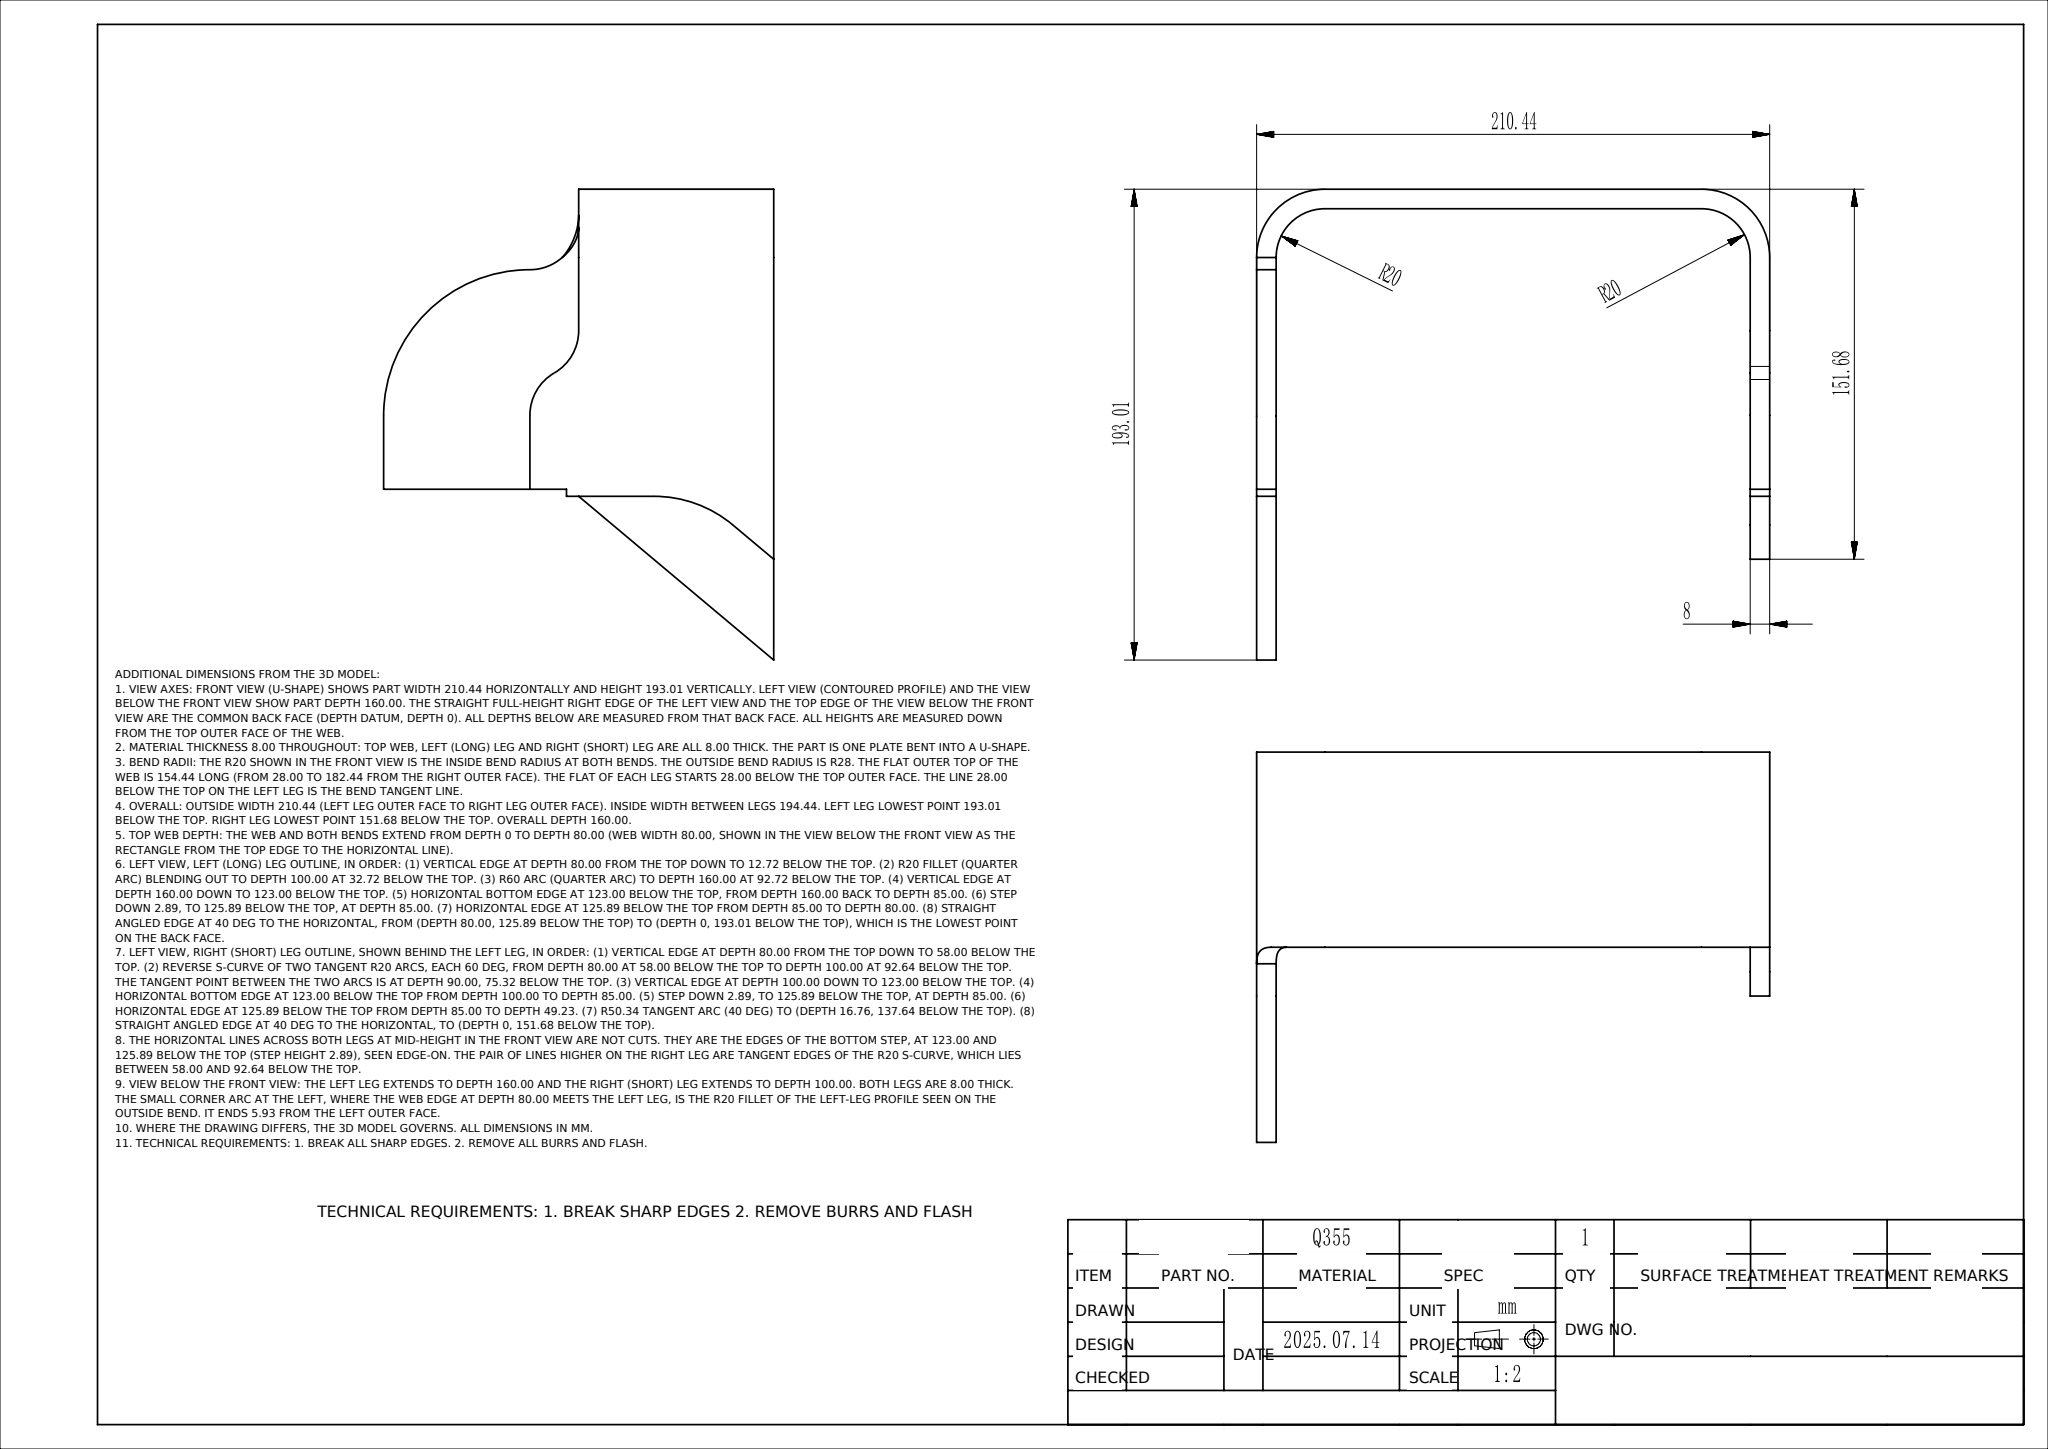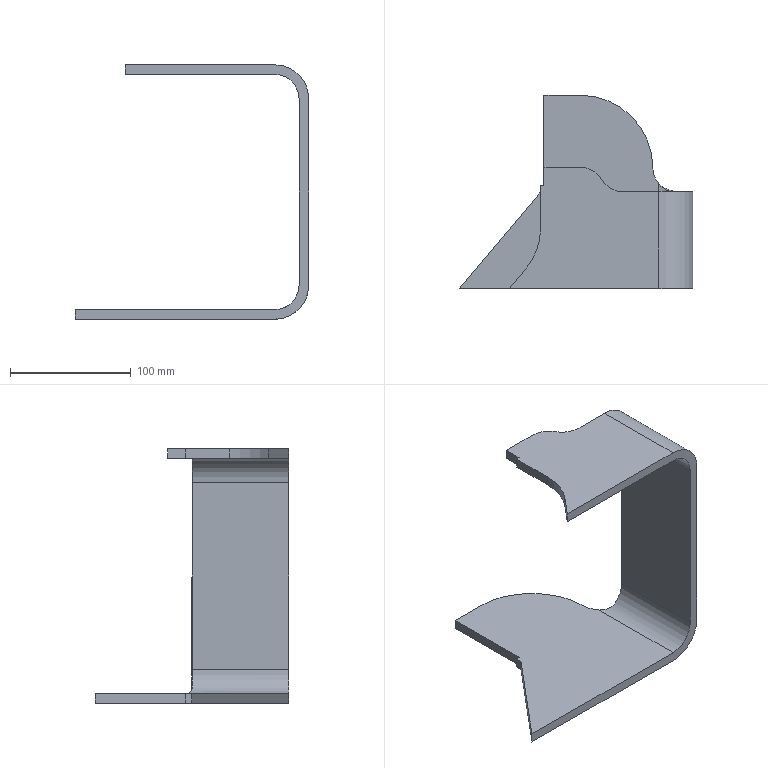Part | NX | mm | 1 solid | 28 faces | box 193.01 x 160 x 210.44 mm | volume 357331 mm3 | plane 18 | cylinder 9 | spline 1 | commonest cylinder face diameters 40 x5 56 x2 120 x1 100.67 x1
STEP:
#1=CARTESIAN_POINT('',(0.,0.,0.));
#2=DIRECTION('',(0.,0.,1.));
#3=DIRECTION('',(1.,0.,0.));
#4=AXIS2_PLACEMENT_3D('',#1,#2,#3);
#5=(LENGTH_UNIT()NAMED_UNIT(*)SI_UNIT(.MILLI.,.METRE.));
#6=UNCERTAINTY_MEASURE_WITH_UNIT(LENGTH_MEASURE(0.0508),#5,'','');
#7=(NAMED_UNIT(*)PLANE_ANGLE_UNIT()SI_UNIT($,.RADIAN.));
#8=PLANE_ANGLE_MEASURE_WITH_UNIT(PLANE_ANGLE_MEASURE(0.01745),#7);
#9=DIMENSIONAL_EXPONENTS(0.,0.,0.,0.,0.,0.,0.);
#10=(CONVERSION_BASED_UNIT('',#8)NAMED_UNIT(#9)PLANE_ANGLE_UNIT());
#11=(NAMED_UNIT(*)SI_UNIT($,.STERADIAN.)SOLID_ANGLE_UNIT());
#12=(GEOMETRIC_REPRESENTATION_CONTEXT(3)GLOBAL_UNCERTAINTY_ASSIGNED_CONTEXT((#6))GLOBAL_UNIT_ASSIGNED_CONTEXT((#5,#10,#11))REPRESENTATION_CONTEXT('',''));
#13=SHAPE_REPRESENTATION('',(#4),#12);
#14=CARTESIAN_POINT('',(123.,-85.,-28.));
#15=VERTEX_POINT('',#14);
#16=CARTESIAN_POINT('',(123.,-85.,-182.437));
#17=VERTEX_POINT('',#16);
#18=CARTESIAN_POINT('',(123.,-85.,131.244));
#19=DIRECTION('',(0.,0.,-1.));
#20=VECTOR('',#19,1.);
#21=LINE('',#18,#20);
#22=EDGE_CURVE('',#15,#17,#21,.T.);
#23=ORIENTED_EDGE('',*,*,#22,.F.);
#24=CARTESIAN_POINT('',(95.,-85.,0.));
#25=VERTEX_POINT('',#24);
#26=CARTESIAN_POINT('',(95.,-85.,-28.));
#27=DIRECTION('',(0.,1.,0.));
#28=DIRECTION('',(0.,0.,-1.));
#29=AXIS2_PLACEMENT_3D('',#26,#27,#28);
#30=CIRCLE('',#29,28.);
#31=EDGE_CURVE('',#25,#15,#30,.T.);
#32=ORIENTED_EDGE('',*,*,#31,.F.);
#33=CARTESIAN_POINT('',(-28.681,-85.,0.));
#34=VERTEX_POINT('',#33);
#35=CARTESIAN_POINT('',(-28.681,-85.,0.));
#36=DIRECTION('',(1.,0.,0.));
#37=VECTOR('',#36,1.);
#38=LINE('',#35,#37);
#39=EDGE_CURVE('',#34,#25,#38,.T.);
#40=ORIENTED_EDGE('',*,*,#39,.F.);
#41=CARTESIAN_POINT('',(-28.681,-85.,-8.));
#42=VERTEX_POINT('',#41);
#43=CARTESIAN_POINT('',(-28.681,-85.,-8.));
#44=DIRECTION('',(0.,0.,1.));
#45=VECTOR('',#44,1.);
#46=LINE('',#43,#45);
#47=EDGE_CURVE('',#42,#34,#46,.T.);
#48=ORIENTED_EDGE('',*,*,#47,.F.);
#49=CARTESIAN_POINT('',(95.,-85.,-8.));
#50=VERTEX_POINT('',#49);
#51=CARTESIAN_POINT('',(-28.681,-85.,-8.));
#52=DIRECTION('',(1.,0.,0.));
#53=VECTOR('',#52,1.);
#54=LINE('',#51,#53);
#55=EDGE_CURVE('',#42,#50,#54,.T.);
#56=ORIENTED_EDGE('',*,*,#55,.T.);
#57=CARTESIAN_POINT('',(115.,-85.,-28.));
#58=VERTEX_POINT('',#57);
#59=CARTESIAN_POINT('',(95.,-85.,-28.));
#60=DIRECTION('',(0.,1.,0.));
#61=DIRECTION('',(0.,0.,1.));
#62=AXIS2_PLACEMENT_3D('',#59,#60,#61);
#63=CIRCLE('',#62,20.);
#64=EDGE_CURVE('',#50,#58,#63,.T.);
#65=ORIENTED_EDGE('',*,*,#64,.T.);
#66=CARTESIAN_POINT('',(115.,-85.,-182.437));
#67=VERTEX_POINT('',#66);
#68=CARTESIAN_POINT('',(115.,-85.,131.244));
#69=DIRECTION('',(0.,0.,-1.));
#70=VECTOR('',#69,1.);
#71=LINE('',#68,#70);
#72=EDGE_CURVE('',#58,#67,#71,.T.);
#73=ORIENTED_EDGE('',*,*,#72,.T.);
#74=CARTESIAN_POINT('',(95.,-85.,-202.437));
#75=VERTEX_POINT('',#74);
#76=CARTESIAN_POINT('',(95.,-85.,-182.437));
#77=DIRECTION('',(0.,1.,0.));
#78=DIRECTION('',(1.,0.,0.));
#79=AXIS2_PLACEMENT_3D('',#76,#77,#78);
#80=CIRCLE('',#79,20.);
#81=EDGE_CURVE('',#67,#75,#80,.T.);
#82=ORIENTED_EDGE('',*,*,#81,.T.);
#83=CARTESIAN_POINT('',(-70.014,-85.,-202.437));
#84=VERTEX_POINT('',#83);
#85=CARTESIAN_POINT('',(444.244,-85.,-202.437));
#86=DIRECTION('',(-1.,0.,-0.));
#87=VECTOR('',#86,1.);
#88=LINE('',#85,#87);
#89=EDGE_CURVE('',#75,#84,#88,.T.);
#90=ORIENTED_EDGE('',*,*,#89,.T.);
#91=CARTESIAN_POINT('',(-70.014,-85.,-210.437));
#92=VERTEX_POINT('',#91);
#93=CARTESIAN_POINT('',(-70.014,-85.,-202.437));
#94=DIRECTION('',(0.,0.,-1.));
#95=VECTOR('',#94,1.);
#96=LINE('',#93,#95);
#97=EDGE_CURVE('',#84,#92,#96,.T.);
#98=ORIENTED_EDGE('',*,*,#97,.T.);
#99=CARTESIAN_POINT('',(95.,-85.,-210.437));
#100=VERTEX_POINT('',#99);
#101=CARTESIAN_POINT('',(444.244,-85.,-210.437));
#102=DIRECTION('',(-1.,0.,-0.));
#103=VECTOR('',#102,1.);
#104=LINE('',#101,#103);
#105=EDGE_CURVE('',#100,#92,#104,.T.);
#106=ORIENTED_EDGE('',*,*,#105,.F.);
#107=CARTESIAN_POINT('',(95.,-85.,-182.437));
#108=DIRECTION('',(0.,1.,0.));
#109=DIRECTION('',(-1.,0.,-0.));
#110=AXIS2_PLACEMENT_3D('',#107,#108,#109);
#111=CIRCLE('',#110,28.);
#112=EDGE_CURVE('',#17,#100,#111,.T.);
#113=ORIENTED_EDGE('',*,*,#112,.F.);
#114=EDGE_LOOP('',(#23,#32,#40,#48,#56,#65,#73,#82,#90,#98,#106,#113));
#115=FACE_OUTER_BOUND('',#114,.T.);
#116=CARTESIAN_POINT('',(444.244,-85.,-202.437));
#117=DIRECTION('',(-0.,-1.,-0.));
#118=DIRECTION('',(-1.,0.,-0.));
#119=AXIS2_PLACEMENT_3D('',#116,#117,#118);
#120=PLANE('',#119);
#121=ADVANCED_FACE('',(#115),#120,.T.);
#122=CARTESIAN_POINT('',(123.,-5.,-182.437));
#123=VERTEX_POINT('',#122);
#124=CARTESIAN_POINT('',(123.,-5.,-28.));
#125=VERTEX_POINT('',#124);
#126=CARTESIAN_POINT('',(123.,-5.,-222.997));
#127=DIRECTION('',(-0.,-0.,1.));
#128=VECTOR('',#127,1.);
#129=LINE('',#126,#128);
#130=EDGE_CURVE('',#123,#125,#129,.T.);
#131=ORIENTED_EDGE('',*,*,#130,.T.);
#132=CARTESIAN_POINT('',(123.,50.,-28.));
#133=DIRECTION('',(0.,-1.,-0.));
#134=VECTOR('',#133,1.);
#135=LINE('',#132,#134);
#136=EDGE_CURVE('',#125,#15,#135,.T.);
#137=ORIENTED_EDGE('',*,*,#136,.T.);
#138=ORIENTED_EDGE('',*,*,#22,.T.);
#139=CARTESIAN_POINT('',(123.,45.151,-182.437));
#140=DIRECTION('',(0.,1.,0.));
#141=VECTOR('',#140,1.);
#142=LINE('',#139,#141);
#143=EDGE_CURVE('',#17,#123,#142,.T.);
#144=ORIENTED_EDGE('',*,*,#143,.T.);
#145=EDGE_LOOP('',(#131,#137,#138,#144));
#146=FACE_OUTER_BOUND('',#145,.T.);
#147=CARTESIAN_POINT('',(123.,-35.915,155.787));
#148=DIRECTION('',(-1.,0.,-0.));
#149=DIRECTION('',(-0.,0.,1.));
#150=AXIS2_PLACEMENT_3D('',#147,#148,#149);
#151=PLANE('',#150);
#152=ADVANCED_FACE('',(#146),#151,.F.);
#153=CARTESIAN_POINT('',(90.003,15.,-210.437));
#154=VERTEX_POINT('',#153);
#155=CARTESIAN_POINT('',(95.,1.774,-210.437));
#156=VERTEX_POINT('',#155);
#157=CARTESIAN_POINT('',(110.003,15.,-210.437));
#158=DIRECTION('',(-0.,0.,1.));
#159=DIRECTION('',(1.,0.,0.));
#160=AXIS2_PLACEMENT_3D('',#157,#158,#159);
#161=CIRCLE('',#160,20.);
#162=EDGE_CURVE('',#154,#156,#161,.T.);
#163=ORIENTED_EDGE('',*,*,#162,.T.);
#164=CARTESIAN_POINT('',(95.,45.151,-210.437));
#165=DIRECTION('',(0.,-1.,0.));
#166=VECTOR('',#165,1.);
#167=LINE('',#164,#166);
#168=EDGE_CURVE('',#156,#100,#167,.T.);
#169=ORIENTED_EDGE('',*,*,#168,.T.);
#170=ORIENTED_EDGE('',*,*,#105,.T.);
#171=CARTESIAN_POINT('',(-2.886,-5.,-210.437));
#172=VERTEX_POINT('',#171);
#173=CARTESIAN_POINT('',(-70.014,-85.,-210.437));
#174=DIRECTION('',(0.6428,0.766,0.));
#175=VECTOR('',#174,1.);
#176=LINE('',#173,#175);
#177=EDGE_CURVE('',#92,#172,#176,.T.);
#178=ORIENTED_EDGE('',*,*,#177,.T.);
#179=CARTESIAN_POINT('',(-2.886,0.,-210.437));
#180=VERTEX_POINT('',#179);
#181=CARTESIAN_POINT('',(-2.886,-5.,-210.437));
#182=DIRECTION('',(0.,1.,0.));
#183=VECTOR('',#182,1.);
#184=LINE('',#181,#183);
#185=EDGE_CURVE('',#172,#180,#184,.T.);
#186=ORIENTED_EDGE('',*,*,#185,.T.);
#187=CARTESIAN_POINT('',(0.002829,0.,-210.437));
#188=VERTEX_POINT('',#187);
#189=CARTESIAN_POINT('',(-2.886,0.,-210.437));
#190=DIRECTION('',(1.,-0.,0.));
#191=VECTOR('',#190,1.);
#192=LINE('',#189,#191);
#193=EDGE_CURVE('',#180,#188,#192,.T.);
#194=ORIENTED_EDGE('',*,*,#193,.T.);
#195=CARTESIAN_POINT('',(0.002829,75.,-210.437));
#196=VERTEX_POINT('',#195);
#197=CARTESIAN_POINT('',(0.002829,0.,-210.437));
#198=DIRECTION('',(0.,1.,0.));
#199=VECTOR('',#198,1.);
#200=LINE('',#197,#199);
#201=EDGE_CURVE('',#188,#196,#200,.T.);
#202=ORIENTED_EDGE('',*,*,#201,.T.);
#203=CARTESIAN_POINT('',(30.003,75.,-210.437));
#204=VERTEX_POINT('',#203);
#205=CARTESIAN_POINT('',(0.002829,75.,-210.437));
#206=DIRECTION('',(1.,-0.,0.));
#207=VECTOR('',#206,1.);
#208=LINE('',#205,#207);
#209=EDGE_CURVE('',#196,#204,#208,.T.);
#210=ORIENTED_EDGE('',*,*,#209,.T.);
#211=CARTESIAN_POINT('',(30.003,15.,-210.437));
#212=DIRECTION('',(0.,0.,-1.));
#213=DIRECTION('',(1.,0.,0.));
#214=AXIS2_PLACEMENT_3D('',#211,#212,#213);
#215=CIRCLE('',#214,60.);
#216=EDGE_CURVE('',#204,#154,#215,.T.);
#217=ORIENTED_EDGE('',*,*,#216,.T.);
#218=EDGE_LOOP('',(#163,#169,#170,#178,#186,#194,#202,#210,#217));
#219=FACE_OUTER_BOUND('',#218,.T.);
#220=CARTESIAN_POINT('',(468.787,-35.915,-210.437));
#221=DIRECTION('',(-0.,0.,1.));
#222=DIRECTION('',(1.,0.,0.));
#223=AXIS2_PLACEMENT_3D('',#220,#221,#222);
#224=PLANE('',#223);
#225=ADVANCED_FACE('',(#219),#224,.F.);
#226=ORIENTED_EDGE('',*,*,#177,.F.);
#227=ORIENTED_EDGE('',*,*,#97,.F.);
#228=CARTESIAN_POINT('',(-2.886,-5.,-202.437));
#229=VERTEX_POINT('',#228);
#230=CARTESIAN_POINT('',(-70.014,-85.,-202.437));
#231=DIRECTION('',(0.6428,0.766,0.));
#232=VECTOR('',#231,1.);
#233=LINE('',#230,#232);
#234=EDGE_CURVE('',#84,#229,#233,.T.);
#235=ORIENTED_EDGE('',*,*,#234,.T.);
#236=CARTESIAN_POINT('',(-2.886,-5.,-202.437));
#237=DIRECTION('',(0.,0.,-1.));
#238=VECTOR('',#237,1.);
#239=LINE('',#236,#238);
#240=EDGE_CURVE('',#229,#172,#239,.T.);
#241=ORIENTED_EDGE('',*,*,#240,.T.);
#242=EDGE_LOOP('',(#226,#227,#235,#241));
#243=FACE_OUTER_BOUND('',#242,.T.);
#244=CARTESIAN_POINT('',(-70.014,-85.,-202.437));
#245=DIRECTION('',(-0.766,0.6428,-0.));
#246=DIRECTION('',(0.6428,0.766,0.));
#247=AXIS2_PLACEMENT_3D('',#244,#245,#246);
#248=PLANE('',#247);
#249=ADVANCED_FACE('',(#243),#248,.T.);
#250=ORIENTED_EDGE('',*,*,#185,.F.);
#251=ORIENTED_EDGE('',*,*,#240,.F.);
#252=CARTESIAN_POINT('',(-2.886,0.,-202.437));
#253=VERTEX_POINT('',#252);
#254=CARTESIAN_POINT('',(-2.886,-5.,-202.437));
#255=DIRECTION('',(0.,1.,0.));
#256=VECTOR('',#255,1.);
#257=LINE('',#254,#256);
#258=EDGE_CURVE('',#229,#253,#257,.T.);
#259=ORIENTED_EDGE('',*,*,#258,.T.);
#260=CARTESIAN_POINT('',(-2.886,0.,-202.437));
#261=DIRECTION('',(0.,0.,-1.));
#262=VECTOR('',#261,1.);
#263=LINE('',#260,#262);
#264=EDGE_CURVE('',#253,#180,#263,.T.);
#265=ORIENTED_EDGE('',*,*,#264,.T.);
#266=EDGE_LOOP('',(#250,#251,#259,#265));
#267=FACE_OUTER_BOUND('',#266,.T.);
#268=CARTESIAN_POINT('',(-2.886,-5.,-202.437));
#269=DIRECTION('',(-1.,0.,-0.));
#270=DIRECTION('',(-0.,0.,1.));
#271=AXIS2_PLACEMENT_3D('',#268,#269,#270);
#272=PLANE('',#271);
#273=ADVANCED_FACE('',(#267),#272,.T.);
#274=ORIENTED_EDGE('',*,*,#193,.F.);
#275=ORIENTED_EDGE('',*,*,#264,.F.);
#276=CARTESIAN_POINT('',(0.002829,0.,-202.437));
#277=VERTEX_POINT('',#276);
#278=CARTESIAN_POINT('',(-2.886,0.,-202.437));
#279=DIRECTION('',(1.,-0.,0.));
#280=VECTOR('',#279,1.);
#281=LINE('',#278,#280);
#282=EDGE_CURVE('',#253,#277,#281,.T.);
#283=ORIENTED_EDGE('',*,*,#282,.T.);
#284=CARTESIAN_POINT('',(0.002829,0.,-202.437));
#285=DIRECTION('',(0.,0.,-1.));
#286=VECTOR('',#285,1.);
#287=LINE('',#284,#286);
#288=EDGE_CURVE('',#277,#188,#287,.T.);
#289=ORIENTED_EDGE('',*,*,#288,.T.);
#290=EDGE_LOOP('',(#274,#275,#283,#289));
#291=FACE_OUTER_BOUND('',#290,.T.);
#292=CARTESIAN_POINT('',(-2.886,0.,-202.437));
#293=DIRECTION('',(0.,1.,0.));
#294=DIRECTION('',(1.,-0.,0.));
#295=AXIS2_PLACEMENT_3D('',#292,#293,#294);
#296=PLANE('',#295);
#297=ADVANCED_FACE('',(#291),#296,.T.);
#298=ORIENTED_EDGE('',*,*,#201,.F.);
#299=ORIENTED_EDGE('',*,*,#288,.F.);
#300=CARTESIAN_POINT('',(0.002829,75.,-202.437));
#301=VERTEX_POINT('',#300);
#302=CARTESIAN_POINT('',(0.002829,0.,-202.437));
#303=DIRECTION('',(0.,1.,0.));
#304=VECTOR('',#303,1.);
#305=LINE('',#302,#304);
#306=EDGE_CURVE('',#277,#301,#305,.T.);
#307=ORIENTED_EDGE('',*,*,#306,.T.);
#308=CARTESIAN_POINT('',(0.002829,75.,-202.437));
#309=DIRECTION('',(0.,0.,-1.));
#310=VECTOR('',#309,1.);
#311=LINE('',#308,#310);
#312=EDGE_CURVE('',#301,#196,#311,.T.);
#313=ORIENTED_EDGE('',*,*,#312,.T.);
#314=EDGE_LOOP('',(#298,#299,#307,#313));
#315=FACE_OUTER_BOUND('',#314,.T.);
#316=CARTESIAN_POINT('',(0.002829,0.,-202.437));
#317=DIRECTION('',(-1.,0.,-0.));
#318=DIRECTION('',(-0.,0.,1.));
#319=AXIS2_PLACEMENT_3D('',#316,#317,#318);
#320=PLANE('',#319);
#321=ADVANCED_FACE('',(#315),#320,.T.);
#322=CARTESIAN_POINT('',(30.003,75.,-202.437));
#323=VERTEX_POINT('',#322);
#324=CARTESIAN_POINT('',(0.002829,75.,-202.437));
#325=DIRECTION('',(1.,-0.,0.));
#326=VECTOR('',#325,1.);
#327=LINE('',#324,#326);
#328=EDGE_CURVE('',#301,#323,#327,.T.);
#329=ORIENTED_EDGE('',*,*,#328,.T.);
#330=CARTESIAN_POINT('',(30.003,75.,-202.437));
#331=DIRECTION('',(0.,0.,-1.));
#332=VECTOR('',#331,1.);
#333=LINE('',#330,#332);
#334=EDGE_CURVE('',#323,#204,#333,.T.);
#335=ORIENTED_EDGE('',*,*,#334,.T.);
#336=ORIENTED_EDGE('',*,*,#209,.F.);
#337=ORIENTED_EDGE('',*,*,#312,.F.);
#338=EDGE_LOOP('',(#329,#335,#336,#337));
#339=FACE_OUTER_BOUND('',#338,.T.);
#340=CARTESIAN_POINT('',(0.002829,75.,-202.437));
#341=DIRECTION('',(0.,1.,0.));
#342=DIRECTION('',(1.,-0.,0.));
#343=AXIS2_PLACEMENT_3D('',#340,#341,#342);
#344=PLANE('',#343);
#345=ADVANCED_FACE('',(#339),#344,.T.);
#346=CARTESIAN_POINT('',(95.,1.774,-202.437));
#347=VERTEX_POINT('',#346);
#348=CARTESIAN_POINT('',(95.,45.151,-202.437));
#349=DIRECTION('',(0.,1.,0.));
#350=VECTOR('',#349,1.);
#351=LINE('',#348,#350);
#352=EDGE_CURVE('',#75,#347,#351,.T.);
#353=ORIENTED_EDGE('',*,*,#352,.T.);
#354=CARTESIAN_POINT('',(90.003,15.,-202.437));
#355=VERTEX_POINT('',#354);
#356=CARTESIAN_POINT('',(110.003,15.,-202.437));
#357=DIRECTION('',(0.,0.,-1.));
#358=DIRECTION('',(1.,0.,0.));
#359=AXIS2_PLACEMENT_3D('',#356,#357,#358);
#360=CIRCLE('',#359,20.);
#361=EDGE_CURVE('',#347,#355,#360,.T.);
#362=ORIENTED_EDGE('',*,*,#361,.T.);
#363=CARTESIAN_POINT('',(30.003,15.,-202.437));
#364=DIRECTION('',(-0.,0.,1.));
#365=DIRECTION('',(1.,0.,0.));
#366=AXIS2_PLACEMENT_3D('',#363,#364,#365);
#367=CIRCLE('',#366,60.);
#368=EDGE_CURVE('',#355,#323,#367,.T.);
#369=ORIENTED_EDGE('',*,*,#368,.T.);
#370=ORIENTED_EDGE('',*,*,#328,.F.);
#371=ORIENTED_EDGE('',*,*,#306,.F.);
#372=ORIENTED_EDGE('',*,*,#282,.F.);
#373=ORIENTED_EDGE('',*,*,#258,.F.);
#374=ORIENTED_EDGE('',*,*,#234,.F.);
#375=ORIENTED_EDGE('',*,*,#89,.F.);
#376=EDGE_LOOP('',(#353,#362,#369,#370,#371,#372,#373,#374,#375));
#377=FACE_OUTER_BOUND('',#376,.T.);
#378=CARTESIAN_POINT('',(468.787,-35.915,-202.437));
#379=DIRECTION('',(-0.,0.,1.));
#380=DIRECTION('',(1.,0.,0.));
#381=AXIS2_PLACEMENT_3D('',#378,#379,#380);
#382=PLANE('',#381);
#383=ADVANCED_FACE('',(#377),#382,.T.);
#384=CARTESIAN_POINT('',(95.,1.774,-210.437));
#385=DIRECTION('',(0.,0.,-1.));
#386=VECTOR('',#385,1.);
#387=LINE('',#384,#386);
#388=EDGE_CURVE('',#347,#156,#387,.T.);
#389=ORIENTED_EDGE('',*,*,#388,.T.);
#390=ORIENTED_EDGE('',*,*,#162,.F.);
#391=CARTESIAN_POINT('',(90.003,15.,-210.437));
#392=DIRECTION('',(0.,0.,-1.));
#393=VECTOR('',#392,1.);
#394=LINE('',#391,#393);
#395=EDGE_CURVE('',#355,#154,#394,.T.);
#396=ORIENTED_EDGE('',*,*,#395,.F.);
#397=ORIENTED_EDGE('',*,*,#361,.F.);
#398=EDGE_LOOP('',(#389,#390,#396,#397));
#399=FACE_OUTER_BOUND('',#398,.T.);
#400=CARTESIAN_POINT('',(110.003,15.,-202.437));
#401=DIRECTION('',(-0.,0.,1.));
#402=DIRECTION('',(1.,0.,0.));
#403=AXIS2_PLACEMENT_3D('',#400,#401,#402);
#404=CYLINDRICAL_SURFACE('',#403,20.);
#405=ADVANCED_FACE('',(#399),#404,.F.);
#406=ORIENTED_EDGE('',*,*,#368,.F.);
#407=ORIENTED_EDGE('',*,*,#395,.T.);
#408=ORIENTED_EDGE('',*,*,#216,.F.);
#409=ORIENTED_EDGE('',*,*,#334,.F.);
#410=EDGE_LOOP('',(#406,#407,#408,#409));
#411=FACE_OUTER_BOUND('',#410,.T.);
#412=CARTESIAN_POINT('',(30.003,15.,-202.437));
#413=DIRECTION('',(0.,0.,-1.));
#414=DIRECTION('',(-1.,0.,-0.));
#415=AXIS2_PLACEMENT_3D('',#412,#413,#414);
#416=CYLINDRICAL_SURFACE('',#415,60.);
#417=ADVANCED_FACE('',(#411),#416,.T.);
#418=CARTESIAN_POINT('',(115.,-5.,-182.437));
#419=VERTEX_POINT('',#418);
#420=CARTESIAN_POINT('',(115.,-5.,-28.));
#421=VERTEX_POINT('',#420);
#422=CARTESIAN_POINT('',(115.,-5.,-222.997));
#423=DIRECTION('',(-0.,-0.,1.));
#424=VECTOR('',#423,1.);
#425=LINE('',#422,#424);
#426=EDGE_CURVE('',#419,#421,#425,.T.);
#427=ORIENTED_EDGE('',*,*,#426,.T.);
#428=CARTESIAN_POINT('',(95.,-5.,-8.));
#429=VERTEX_POINT('',#428);
#430=CARTESIAN_POINT('',(95.,-5.,-28.));
#431=DIRECTION('',(0.,-1.,0.));
#432=DIRECTION('',(0.,0.,1.));
#433=AXIS2_PLACEMENT_3D('',#430,#431,#432);
#434=CIRCLE('',#433,20.);
#435=EDGE_CURVE('',#421,#429,#434,.T.);
#436=ORIENTED_EDGE('',*,*,#435,.T.);
#437=CARTESIAN_POINT('',(65.,-5.,-8.));
#438=VERTEX_POINT('',#437);
#439=CARTESIAN_POINT('',(325.56,-5.,-8.));
#440=DIRECTION('',(-1.,-0.,0.));
#441=VECTOR('',#440,1.);
#442=LINE('',#439,#441);
#443=EDGE_CURVE('',#429,#438,#442,.T.);
#444=ORIENTED_EDGE('',*,*,#443,.T.);
#445=CARTESIAN_POINT('',(65.,-5.,0.));
#446=VERTEX_POINT('',#445);
#447=CARTESIAN_POINT('',(65.,-5.,0.));
#448=DIRECTION('',(0.,0.,1.));
#449=VECTOR('',#448,1.);
#450=LINE('',#447,#449);
#451=EDGE_CURVE('',#438,#446,#450,.T.);
#452=ORIENTED_EDGE('',*,*,#451,.T.);
#453=CARTESIAN_POINT('',(95.,-5.,0.));
#454=VERTEX_POINT('',#453);
#455=CARTESIAN_POINT('',(325.56,-5.,0.));
#456=DIRECTION('',(-1.,-0.,0.));
#457=VECTOR('',#456,1.);
#458=LINE('',#455,#457);
#459=EDGE_CURVE('',#454,#446,#458,.T.);
#460=ORIENTED_EDGE('',*,*,#459,.F.);
#461=CARTESIAN_POINT('',(95.,-5.,-28.));
#462=DIRECTION('',(0.,-1.,0.));
#463=DIRECTION('',(0.,0.,-1.));
#464=AXIS2_PLACEMENT_3D('',#461,#462,#463);
#465=CIRCLE('',#464,28.);
#466=EDGE_CURVE('',#125,#454,#465,.T.);
#467=ORIENTED_EDGE('',*,*,#466,.F.);
#468=ORIENTED_EDGE('',*,*,#130,.F.);
#469=CARTESIAN_POINT('',(112.226,-5.,-204.511));
#470=VERTEX_POINT('',#469);
#471=CARTESIAN_POINT('',(95.,-5.,-182.437));
#472=DIRECTION('',(0.,-1.,0.));
#473=DIRECTION('',(-1.,0.,-0.));
#474=AXIS2_PLACEMENT_3D('',#471,#472,#473);
#475=CIRCLE('',#474,28.);
#476=EDGE_CURVE('',#470,#123,#475,.T.);
#477=ORIENTED_EDGE('',*,*,#476,.F.);
#478=CARTESIAN_POINT('',(107.304,-5.,-198.204));
#479=VERTEX_POINT('',#478);
#480=CARTESIAN_POINT('',(112.226,-5.,-204.511));
#481=DIRECTION('',(0.6152,0.,-0.7884));
#482=VECTOR('',#481,1.);
#483=LINE('',#480,#482);
#484=EDGE_CURVE('',#479,#470,#483,.T.);
#485=ORIENTED_EDGE('',*,*,#484,.F.);
#486=CARTESIAN_POINT('',(95.,-5.,-182.437));
#487=DIRECTION('',(0.,-1.,0.));
#488=DIRECTION('',(1.,0.,0.));
#489=AXIS2_PLACEMENT_3D('',#486,#487,#488);
#490=CIRCLE('',#489,20.);
#491=EDGE_CURVE('',#479,#419,#490,.T.);
#492=ORIENTED_EDGE('',*,*,#491,.T.);
#493=EDGE_LOOP('',(#427,#436,#444,#452,#460,#467,#468,#477,#485,#492));
#494=FACE_OUTER_BOUND('',#493,.T.);
#495=CARTESIAN_POINT('',(115.,-5.,-222.997));
#496=DIRECTION('',(-0.,1.,0.));
#497=DIRECTION('',(-0.,-0.,1.));
#498=AXIS2_PLACEMENT_3D('',#495,#496,#497);
#499=PLANE('',#498);
#500=ADVANCED_FACE('',(#494),#499,.T.);
#501=CARTESIAN_POINT('',(115.,50.,-28.));
#502=DIRECTION('',(-0.,1.,0.));
#503=VECTOR('',#502,1.);
#504=LINE('',#501,#503);
#505=EDGE_CURVE('',#58,#421,#504,.T.);
#506=ORIENTED_EDGE('',*,*,#505,.T.);
#507=ORIENTED_EDGE('',*,*,#426,.F.);
#508=CARTESIAN_POINT('',(115.,45.151,-182.437));
#509=DIRECTION('',(0.,-1.,0.));
#510=VECTOR('',#509,1.);
#511=LINE('',#508,#510);
#512=EDGE_CURVE('',#419,#67,#511,.T.);
#513=ORIENTED_EDGE('',*,*,#512,.T.);
#514=ORIENTED_EDGE('',*,*,#72,.F.);
#515=EDGE_LOOP('',(#506,#507,#513,#514));
#516=FACE_OUTER_BOUND('',#515,.T.);
#517=CARTESIAN_POINT('',(115.,-35.915,155.787));
#518=DIRECTION('',(-1.,0.,-0.));
#519=DIRECTION('',(-0.,0.,1.));
#520=AXIS2_PLACEMENT_3D('',#517,#518,#519);
#521=PLANE('',#520);
#522=ADVANCED_FACE('',(#516),#521,.T.);
#523=ORIENTED_EDGE('',*,*,#388,.F.);
#524=CARTESIAN_POINT('',(95.,1.774,-202.437));
#525=CARTESIAN_POINT('',(95.826,0.7141,-202.437));
#526=CARTESIAN_POINT('',(96.752,-0.2471,-202.386));
#527=CARTESIAN_POINT('',(98.742,-1.927,-202.11));
#528=CARTESIAN_POINT('',(99.806,-2.646,-201.885));
#529=CARTESIAN_POINT('',(101.981,-3.81,-201.214));
#530=CARTESIAN_POINT('',(103.093,-4.254,-200.767));
#531=CARTESIAN_POINT('',(104.72,-4.701,-199.927));
#532=CARTESIAN_POINT('',(105.256,-4.813,-199.619));
#533=CARTESIAN_POINT('',(106.302,-4.962,-198.949));
#534=CARTESIAN_POINT('',(106.812,-5.,-198.588));
#535=CARTESIAN_POINT('',(107.304,-5.,-198.204));
#536=B_SPLINE_CURVE_WITH_KNOTS('',3,(#524,#525,#526,#527,#528,#529,#530,#531,#532,#533,#534,#535),.UNSPECIFIED.,.F.,.F.,(4,2,2,2,2,4),(0.,0.25,0.5,0.75,0.875,1.),.UNSPECIFIED.);
#537=EDGE_CURVE('',#347,#479,#536,.T.);
#538=ORIENTED_EDGE('',*,*,#537,.T.);
#539=ORIENTED_EDGE('',*,*,#484,.T.);
#540=CARTESIAN_POINT('',(95.,1.774,-210.437));
#541=CARTESIAN_POINT('',(97.312,-0.3466,-210.437));
#542=CARTESIAN_POINT('',(100.205,-2.064,-210.133));
#543=CARTESIAN_POINT('',(106.297,-4.392,-208.255));
#544=CARTESIAN_POINT('',(109.469,-5.,-206.662));
#545=CARTESIAN_POINT('',(112.226,-5.,-204.511));
#546=B_SPLINE_CURVE_WITH_KNOTS('',3,(#540,#541,#542,#543,#544,#545),.UNSPECIFIED.,.F.,.F.,(4,2,4),(0.,0.5,1.),.UNSPECIFIED.);
#547=EDGE_CURVE('',#156,#470,#546,.T.);
#548=ORIENTED_EDGE('',*,*,#547,.F.);
#549=EDGE_LOOP('',(#523,#538,#539,#548));
#550=FACE_OUTER_BOUND('',#549,.T.);
#551=CARTESIAN_POINT('',(95.,1.774,-210.437));
#552=CARTESIAN_POINT('',(96.156,0.7141,-210.437));
#553=CARTESIAN_POINT('',(97.453,-0.2471,-210.365));
#554=CARTESIAN_POINT('',(100.239,-1.927,-209.979));
#555=CARTESIAN_POINT('',(101.728,-2.646,-209.663));
#556=CARTESIAN_POINT('',(104.774,-3.81,-208.724));
#557=CARTESIAN_POINT('',(106.33,-4.254,-208.1));
#558=CARTESIAN_POINT('',(108.608,-4.701,-206.923));
#559=CARTESIAN_POINT('',(109.358,-4.813,-206.491));
#560=CARTESIAN_POINT('',(110.823,-4.962,-205.554));
#561=CARTESIAN_POINT('',(111.537,-5.,-205.049));
#562=CARTESIAN_POINT('',(112.226,-5.,-204.511));
#563=CARTESIAN_POINT('',(95.,1.774,-202.437));
#564=CARTESIAN_POINT('',(95.826,0.7141,-202.437));
#565=CARTESIAN_POINT('',(96.752,-0.2471,-202.386));
#566=CARTESIAN_POINT('',(98.742,-1.927,-202.11));
#567=CARTESIAN_POINT('',(99.806,-2.646,-201.885));
#568=CARTESIAN_POINT('',(101.981,-3.81,-201.214));
#569=CARTESIAN_POINT('',(103.093,-4.254,-200.767));
#570=CARTESIAN_POINT('',(104.72,-4.701,-199.927));
#571=CARTESIAN_POINT('',(105.256,-4.813,-199.619));
#572=CARTESIAN_POINT('',(106.302,-4.962,-198.949));
#573=CARTESIAN_POINT('',(106.812,-5.,-198.588));
#574=CARTESIAN_POINT('',(107.304,-5.,-198.204));
#575=B_SPLINE_SURFACE_WITH_KNOTS('',1,3,((#551,#552,#553,#554,#555,#556,#557,#558,#559,#560,#561,#562),(#563,#564,#565,#566,#567,#568,#569,#570,#571,#572,#573,#574)),.UNSPECIFIED.,.F.,.F.,.F.,(2,2),(4,2,2,2,2,4),(0.,1.),(0.,0.25,0.5,0.75,0.875,1.),.UNSPECIFIED.);
#576=ADVANCED_FACE('',(#550),#575,.T.);
#577=ORIENTED_EDGE('',*,*,#112,.T.);
#578=ORIENTED_EDGE('',*,*,#168,.F.);
#579=ORIENTED_EDGE('',*,*,#547,.T.);
#580=ORIENTED_EDGE('',*,*,#476,.T.);
#581=ORIENTED_EDGE('',*,*,#143,.F.);
#582=EDGE_LOOP('',(#577,#578,#579,#580,#581));
#583=FACE_OUTER_BOUND('',#582,.T.);
#584=CARTESIAN_POINT('',(95.,-85.,-182.437));
#585=DIRECTION('',(0.,1.,0.));
#586=DIRECTION('',(-1.,0.,-0.));
#587=AXIS2_PLACEMENT_3D('',#584,#585,#586);
#588=CYLINDRICAL_SURFACE('',#587,28.);
#589=ADVANCED_FACE('',(#583),#588,.T.);
#590=ORIENTED_EDGE('',*,*,#81,.F.);
#591=ORIENTED_EDGE('',*,*,#512,.F.);
#592=ORIENTED_EDGE('',*,*,#491,.F.);
#593=ORIENTED_EDGE('',*,*,#537,.F.);
#594=ORIENTED_EDGE('',*,*,#352,.F.);
#595=EDGE_LOOP('',(#590,#591,#592,#593,#594));
#596=FACE_OUTER_BOUND('',#595,.T.);
#597=CARTESIAN_POINT('',(95.,-85.,-182.437));
#598=DIRECTION('',(0.,1.,0.));
#599=DIRECTION('',(-1.,0.,-0.));
#600=AXIS2_PLACEMENT_3D('',#597,#598,#599);
#601=CYLINDRICAL_SURFACE('',#600,20.);
#602=ADVANCED_FACE('',(#596),#601,.F.);
#603=CARTESIAN_POINT('',(30.359,15.,-8.));
#604=VERTEX_POINT('',#603);
#605=CARTESIAN_POINT('',(47.679,5.,-8.));
#606=VERTEX_POINT('',#605);
#607=CARTESIAN_POINT('',(30.359,-5.,-8.));
#608=DIRECTION('',(0.,0.,-1.));
#609=DIRECTION('',(-1.,0.,0.));
#610=AXIS2_PLACEMENT_3D('',#607,#608,#609);
#611=CIRCLE('',#610,20.);
#612=EDGE_CURVE('',#604,#606,#611,.T.);
#613=ORIENTED_EDGE('',*,*,#612,.F.);
#614=CARTESIAN_POINT('',(30.359,15.,0.));
#615=VERTEX_POINT('',#614);
#616=CARTESIAN_POINT('',(30.359,15.,-8.));
#617=DIRECTION('',(0.,0.,-1.));
#618=VECTOR('',#617,1.);
#619=LINE('',#616,#618);
#620=EDGE_CURVE('',#615,#604,#619,.T.);
#621=ORIENTED_EDGE('',*,*,#620,.F.);
#622=CARTESIAN_POINT('',(47.679,5.,0.));
#623=VERTEX_POINT('',#622);
#624=CARTESIAN_POINT('',(30.359,-5.,0.));
#625=DIRECTION('',(0.,0.,1.));
#626=DIRECTION('',(-1.,0.,0.));
#627=AXIS2_PLACEMENT_3D('',#624,#625,#626);
#628=CIRCLE('',#627,20.);
#629=EDGE_CURVE('',#623,#615,#628,.T.);
#630=ORIENTED_EDGE('',*,*,#629,.F.);
#631=CARTESIAN_POINT('',(47.679,5.,-8.));
#632=DIRECTION('',(0.,0.,1.));
#633=VECTOR('',#632,1.);
#634=LINE('',#631,#633);
#635=EDGE_CURVE('',#606,#623,#634,.T.);
#636=ORIENTED_EDGE('',*,*,#635,.F.);
#637=EDGE_LOOP('',(#613,#621,#630,#636));
#638=FACE_OUTER_BOUND('',#637,.T.);
#639=CARTESIAN_POINT('',(30.359,-5.,-8.));
#640=DIRECTION('',(0.,0.,-1.));
#641=DIRECTION('',(-1.,0.,0.));
#642=AXIS2_PLACEMENT_3D('',#639,#640,#641);
#643=CYLINDRICAL_SURFACE('',#642,20.);
#644=ADVANCED_FACE('',(#638),#643,.T.);
#645=CARTESIAN_POINT('',(0.,15.,0.));
#646=VERTEX_POINT('',#645);
#647=CARTESIAN_POINT('',(45.,15.,0.));
#648=DIRECTION('',(-1.,0.,0.));
#649=VECTOR('',#648,1.);
#650=LINE('',#647,#649);
#651=EDGE_CURVE('',#615,#646,#650,.T.);
#652=ORIENTED_EDGE('',*,*,#651,.F.);
#653=ORIENTED_EDGE('',*,*,#620,.T.);
#654=CARTESIAN_POINT('',(0.,15.,-8.));
#655=VERTEX_POINT('',#654);
#656=CARTESIAN_POINT('',(45.,15.,-8.));
#657=DIRECTION('',(-1.,0.,0.));
#658=VECTOR('',#657,1.);
#659=LINE('',#656,#658);
#660=EDGE_CURVE('',#604,#655,#659,.T.);
#661=ORIENTED_EDGE('',*,*,#660,.T.);
#662=CARTESIAN_POINT('',(0.,15.,-8.));
#663=DIRECTION('',(0.,0.,1.));
#664=VECTOR('',#663,1.);
#665=LINE('',#662,#664);
#666=EDGE_CURVE('',#655,#646,#665,.T.);
#667=ORIENTED_EDGE('',*,*,#666,.T.);
#668=EDGE_LOOP('',(#652,#653,#661,#667));
#669=FACE_OUTER_BOUND('',#668,.T.);
#670=CARTESIAN_POINT('',(45.,15.,-8.));
#671=DIRECTION('',(0.,1.,0.));
#672=DIRECTION('',(0.,0.,1.));
#673=AXIS2_PLACEMENT_3D('',#670,#671,#672);
#674=PLANE('',#673);
#675=ADVANCED_FACE('',(#669),#674,.T.);
#676=CARTESIAN_POINT('',(0.,0.,0.));
#677=VERTEX_POINT('',#676);
#678=CARTESIAN_POINT('',(0.,15.,0.));
#679=DIRECTION('',(0.,-1.,0.));
#680=VECTOR('',#679,1.);
#681=LINE('',#678,#680);
#682=EDGE_CURVE('',#646,#677,#681,.T.);
#683=ORIENTED_EDGE('',*,*,#682,.F.);
#684=ORIENTED_EDGE('',*,*,#666,.F.);
#685=CARTESIAN_POINT('',(0.,0.,-8.));
#686=VERTEX_POINT('',#685);
#687=CARTESIAN_POINT('',(0.,15.,-8.));
#688=DIRECTION('',(0.,-1.,0.));
#689=VECTOR('',#688,1.);
#690=LINE('',#687,#689);
#691=EDGE_CURVE('',#655,#686,#690,.T.);
#692=ORIENTED_EDGE('',*,*,#691,.T.);
#693=CARTESIAN_POINT('',(0.,0.,-8.));
#694=DIRECTION('',(0.,0.,1.));
#695=VECTOR('',#694,1.);
#696=LINE('',#693,#695);
#697=EDGE_CURVE('',#686,#677,#696,.T.);
#698=ORIENTED_EDGE('',*,*,#697,.T.);
#699=EDGE_LOOP('',(#683,#684,#692,#698));
#700=FACE_OUTER_BOUND('',#699,.T.);
#701=CARTESIAN_POINT('',(0.,15.,-8.));
#702=DIRECTION('',(-1.,0.,0.));
#703=DIRECTION('',(0.,0.,1.));
#704=AXIS2_PLACEMENT_3D('',#701,#702,#703);
#705=PLANE('',#704);
#706=ADVANCED_FACE('',(#700),#705,.T.);
#707=CARTESIAN_POINT('',(-2.889,0.,0.));
#708=VERTEX_POINT('',#707);
#709=CARTESIAN_POINT('',(0.,0.,0.));
#710=DIRECTION('',(-1.,0.,0.));
#711=VECTOR('',#710,1.);
#712=LINE('',#709,#711);
#713=EDGE_CURVE('',#677,#708,#712,.T.);
#714=ORIENTED_EDGE('',*,*,#713,.F.);
#715=ORIENTED_EDGE('',*,*,#697,.F.);
#716=CARTESIAN_POINT('',(-2.889,0.,-8.));
#717=VERTEX_POINT('',#716);
#718=CARTESIAN_POINT('',(0.,0.,-8.));
#719=DIRECTION('',(-1.,0.,0.));
#720=VECTOR('',#719,1.);
#721=LINE('',#718,#720);
#722=EDGE_CURVE('',#686,#717,#721,.T.);
#723=ORIENTED_EDGE('',*,*,#722,.T.);
#724=CARTESIAN_POINT('',(-2.889,0.,-8.));
#725=DIRECTION('',(0.,0.,1.));
#726=VECTOR('',#725,1.);
#727=LINE('',#724,#726);
#728=EDGE_CURVE('',#717,#708,#727,.T.);
#729=ORIENTED_EDGE('',*,*,#728,.T.);
#730=EDGE_LOOP('',(#714,#715,#723,#729));
#731=FACE_OUTER_BOUND('',#730,.T.);
#732=CARTESIAN_POINT('',(0.,0.,-8.));
#733=DIRECTION('',(0.,1.,0.));
#734=DIRECTION('',(0.,0.,1.));
#735=AXIS2_PLACEMENT_3D('',#732,#733,#734);
#736=PLANE('',#735);
#737=ADVANCED_FACE('',(#731),#736,.T.);
#738=CARTESIAN_POINT('',(-2.889,-35.769,0.));
#739=VERTEX_POINT('',#738);
#740=CARTESIAN_POINT('',(-2.889,0.,0.));
#741=DIRECTION('',(-0.,-1.,0.));
#742=VECTOR('',#741,1.);
#743=LINE('',#740,#742);
#744=EDGE_CURVE('',#708,#739,#743,.T.);
#745=ORIENTED_EDGE('',*,*,#744,.F.);
#746=ORIENTED_EDGE('',*,*,#728,.F.);
#747=CARTESIAN_POINT('',(-2.889,-35.769,-8.));
#748=VERTEX_POINT('',#747);
#749=CARTESIAN_POINT('',(-2.889,0.,-8.));
#750=DIRECTION('',(-0.,-1.,0.));
#751=VECTOR('',#750,1.);
#752=LINE('',#749,#751);
#753=EDGE_CURVE('',#717,#748,#752,.T.);
#754=ORIENTED_EDGE('',*,*,#753,.T.);
#755=CARTESIAN_POINT('',(-2.889,-35.769,-8.));
#756=DIRECTION('',(0.,0.,1.));
#757=VECTOR('',#756,1.);
#758=LINE('',#755,#757);
#759=EDGE_CURVE('',#748,#739,#758,.T.);
#760=ORIENTED_EDGE('',*,*,#759,.T.);
#761=EDGE_LOOP('',(#745,#746,#754,#760));
#762=FACE_OUTER_BOUND('',#761,.T.);
#763=CARTESIAN_POINT('',(-2.889,0.,-8.));
#764=DIRECTION('',(-1.,0.,0.));
#765=DIRECTION('',(-0.,-1.,0.));
#766=AXIS2_PLACEMENT_3D('',#763,#764,#765);
#767=PLANE('',#766);
#768=ADVANCED_FACE('',(#762),#767,.T.);
#769=CARTESIAN_POINT('',(-14.64,-68.241,0.));
#770=VERTEX_POINT('',#769);
#771=CARTESIAN_POINT('',(-53.224,-35.915,0.));
#772=DIRECTION('',(0.,0.,-1.));
#773=DIRECTION('',(1.,0.,0.));
#774=AXIS2_PLACEMENT_3D('',#771,#772,#773);
#775=CIRCLE('',#774,50.335);
#776=EDGE_CURVE('',#739,#770,#775,.T.);
#777=ORIENTED_EDGE('',*,*,#776,.F.);
#778=ORIENTED_EDGE('',*,*,#759,.F.);
#779=CARTESIAN_POINT('',(-14.64,-68.241,-8.));
#780=VERTEX_POINT('',#779);
#781=CARTESIAN_POINT('',(-53.224,-35.915,-8.));
#782=DIRECTION('',(0.,0.,-1.));
#783=DIRECTION('',(1.,0.,0.));
#784=AXIS2_PLACEMENT_3D('',#781,#782,#783);
#785=CIRCLE('',#784,50.335);
#786=EDGE_CURVE('',#748,#780,#785,.T.);
#787=ORIENTED_EDGE('',*,*,#786,.T.);
#788=CARTESIAN_POINT('',(-14.64,-68.241,-8.));
#789=DIRECTION('',(0.,0.,1.));
#790=VECTOR('',#789,1.);
#791=LINE('',#788,#790);
#792=EDGE_CURVE('',#780,#770,#791,.T.);
#793=ORIENTED_EDGE('',*,*,#792,.T.);
#794=EDGE_LOOP('',(#777,#778,#787,#793));
#795=FACE_OUTER_BOUND('',#794,.T.);
#796=CARTESIAN_POINT('',(-53.224,-35.915,-8.));
#797=DIRECTION('',(0.,0.,1.));
#798=DIRECTION('',(1.,0.,0.));
#799=AXIS2_PLACEMENT_3D('',#796,#797,#798);
#800=CYLINDRICAL_SURFACE('',#799,50.335);
#801=ADVANCED_FACE('',(#795),#800,.F.);
#802=CARTESIAN_POINT('',(-14.64,-68.241,0.));
#803=DIRECTION('',(-0.6422,-0.7665,0.));
#804=VECTOR('',#803,1.);
#805=LINE('',#802,#804);
#806=EDGE_CURVE('',#770,#34,#805,.T.);
#807=ORIENTED_EDGE('',*,*,#806,.F.);
#808=ORIENTED_EDGE('',*,*,#792,.F.);
#809=CARTESIAN_POINT('',(-14.64,-68.241,-8.));
#810=DIRECTION('',(-0.6422,-0.7665,0.));
#811=VECTOR('',#810,1.);
#812=LINE('',#809,#811);
#813=EDGE_CURVE('',#780,#42,#812,.T.);
#814=ORIENTED_EDGE('',*,*,#813,.T.);
#815=ORIENTED_EDGE('',*,*,#47,.T.);
#816=EDGE_LOOP('',(#807,#808,#814,#815));
#817=FACE_OUTER_BOUND('',#816,.T.);
#818=CARTESIAN_POINT('',(-14.64,-68.241,-8.));
#819=DIRECTION('',(-0.7665,0.6422,0.));
#820=DIRECTION('',(-0.6422,-0.7665,0.));
#821=AXIS2_PLACEMENT_3D('',#818,#819,#820);
#822=PLANE('',#821);
#823=ADVANCED_FACE('',(#817),#822,.T.);
#824=CARTESIAN_POINT('',(65.,15.,-8.));
#825=DIRECTION('',(0.,0.,1.));
#826=DIRECTION('',(-1.,0.,0.));
#827=AXIS2_PLACEMENT_3D('',#824,#825,#826);
#828=CIRCLE('',#827,20.);
#829=EDGE_CURVE('',#606,#438,#828,.T.);
#830=ORIENTED_EDGE('',*,*,#829,.F.);
#831=ORIENTED_EDGE('',*,*,#635,.T.);
#832=CARTESIAN_POINT('',(65.,15.,0.));
#833=DIRECTION('',(0.,0.,-1.));
#834=DIRECTION('',(-1.,0.,0.));
#835=AXIS2_PLACEMENT_3D('',#832,#833,#834);
#836=CIRCLE('',#835,20.);
#837=EDGE_CURVE('',#446,#623,#836,.T.);
#838=ORIENTED_EDGE('',*,*,#837,.F.);
#839=ORIENTED_EDGE('',*,*,#451,.F.);
#840=EDGE_LOOP('',(#830,#831,#838,#839));
#841=FACE_OUTER_BOUND('',#840,.T.);
#842=CARTESIAN_POINT('',(65.,15.,-8.));
#843=DIRECTION('',(0.,0.,-1.));
#844=DIRECTION('',(-1.,0.,0.));
#845=AXIS2_PLACEMENT_3D('',#842,#843,#844);
#846=CYLINDRICAL_SURFACE('',#845,20.);
#847=ADVANCED_FACE('',(#841),#846,.F.);
#848=ORIENTED_EDGE('',*,*,#443,.F.);
#849=CARTESIAN_POINT('',(95.,50.,-8.));
#850=DIRECTION('',(0.,-1.,0.));
#851=VECTOR('',#850,1.);
#852=LINE('',#849,#851);
#853=EDGE_CURVE('',#429,#50,#852,.T.);
#854=ORIENTED_EDGE('',*,*,#853,.T.);
#855=ORIENTED_EDGE('',*,*,#55,.F.);
#856=ORIENTED_EDGE('',*,*,#813,.F.);
#857=ORIENTED_EDGE('',*,*,#786,.F.);
#858=ORIENTED_EDGE('',*,*,#753,.F.);
#859=ORIENTED_EDGE('',*,*,#722,.F.);
#860=ORIENTED_EDGE('',*,*,#691,.F.);
#861=ORIENTED_EDGE('',*,*,#660,.F.);
#862=ORIENTED_EDGE('',*,*,#612,.T.);
#863=ORIENTED_EDGE('',*,*,#829,.T.);
#864=EDGE_LOOP('',(#848,#854,#855,#856,#857,#858,#859,#860,#861,#862,#863));
#865=FACE_OUTER_BOUND('',#864,.T.);
#866=CARTESIAN_POINT('',(-53.224,-35.915,-8.));
#867=DIRECTION('',(0.,0.,-1.));
#868=DIRECTION('',(-1.,0.,0.));
#869=AXIS2_PLACEMENT_3D('',#866,#867,#868);
#870=PLANE('',#869);
#871=ADVANCED_FACE('',(#865),#870,.T.);
#872=CARTESIAN_POINT('',(95.,50.,0.));
#873=DIRECTION('',(-0.,1.,0.));
#874=VECTOR('',#873,1.);
#875=LINE('',#872,#874);
#876=EDGE_CURVE('',#25,#454,#875,.T.);
#877=ORIENTED_EDGE('',*,*,#876,.T.);
#878=ORIENTED_EDGE('',*,*,#459,.T.);
#879=ORIENTED_EDGE('',*,*,#837,.T.);
#880=ORIENTED_EDGE('',*,*,#629,.T.);
#881=ORIENTED_EDGE('',*,*,#651,.T.);
#882=ORIENTED_EDGE('',*,*,#682,.T.);
#883=ORIENTED_EDGE('',*,*,#713,.T.);
#884=ORIENTED_EDGE('',*,*,#744,.T.);
#885=ORIENTED_EDGE('',*,*,#776,.T.);
#886=ORIENTED_EDGE('',*,*,#806,.T.);
#887=ORIENTED_EDGE('',*,*,#39,.T.);
#888=EDGE_LOOP('',(#877,#878,#879,#880,#881,#882,#883,#884,#885,#886,#887));
#889=FACE_OUTER_BOUND('',#888,.T.);
#890=CARTESIAN_POINT('',(-53.224,-35.915,0.));
#891=DIRECTION('',(0.,0.,-1.));
#892=DIRECTION('',(-1.,0.,0.));
#893=AXIS2_PLACEMENT_3D('',#890,#891,#892);
#894=PLANE('',#893);
#895=ADVANCED_FACE('',(#889),#894,.F.);
#896=ORIENTED_EDGE('',*,*,#31,.T.);
#897=ORIENTED_EDGE('',*,*,#136,.F.);
#898=ORIENTED_EDGE('',*,*,#466,.T.);
#899=ORIENTED_EDGE('',*,*,#876,.F.);
#900=EDGE_LOOP('',(#896,#897,#898,#899));
#901=FACE_OUTER_BOUND('',#900,.T.);
#902=CARTESIAN_POINT('',(95.,-85.,-28.));
#903=DIRECTION('',(0.,1.,0.));
#904=DIRECTION('',(0.,0.,-1.));
#905=AXIS2_PLACEMENT_3D('',#902,#903,#904);
#906=CYLINDRICAL_SURFACE('',#905,28.);
#907=ADVANCED_FACE('',(#901),#906,.T.);
#908=ORIENTED_EDGE('',*,*,#64,.F.);
#909=ORIENTED_EDGE('',*,*,#853,.F.);
#910=ORIENTED_EDGE('',*,*,#435,.F.);
#911=ORIENTED_EDGE('',*,*,#505,.F.);
#912=EDGE_LOOP('',(#908,#909,#910,#911));
#913=FACE_OUTER_BOUND('',#912,.T.);
#914=CARTESIAN_POINT('',(95.,-85.,-28.));
#915=DIRECTION('',(0.,1.,0.));
#916=DIRECTION('',(0.,0.,-1.));
#917=AXIS2_PLACEMENT_3D('',#914,#915,#916);
#918=CYLINDRICAL_SURFACE('',#917,20.);
#919=ADVANCED_FACE('',(#913),#918,.F.);
#920=CLOSED_SHELL('',(#121,#152,#225,#249,#273,#297,#321,#345,#383,#405,#417,#500,#522,#576,#589,#602,#644,#675,#706,#737,#768,#801,#823,#847,#871,#895,#907,#919));
#921=MANIFOLD_SOLID_BREP('',#920);
#922=ADVANCED_BREP_SHAPE_REPRESENTATION('',(#921),#12);
#923=SHAPE_REPRESENTATION_RELATIONSHIP('','',#13,#922);
#924=PRESENTATION_LAYER_ASSIGNMENT('','',(#921));
#925=COLOUR_RGB('',0.5961,0.6667,0.6863);
#926=FILL_AREA_STYLE_COLOUR('',#925);
#927=FILL_AREA_STYLE('',(#926));
#928=SURFACE_STYLE_FILL_AREA(#927);
#929=SURFACE_SIDE_STYLE('',(#928));
#930=SURFACE_STYLE_USAGE(.BOTH.,#929);
#931=PRESENTATION_STYLE_ASSIGNMENT((#930));
#932=STYLED_ITEM('',(#931),#921);
#933=MECHANICAL_DESIGN_GEOMETRIC_PRESENTATION_REPRESENTATION('',(#932),#12);